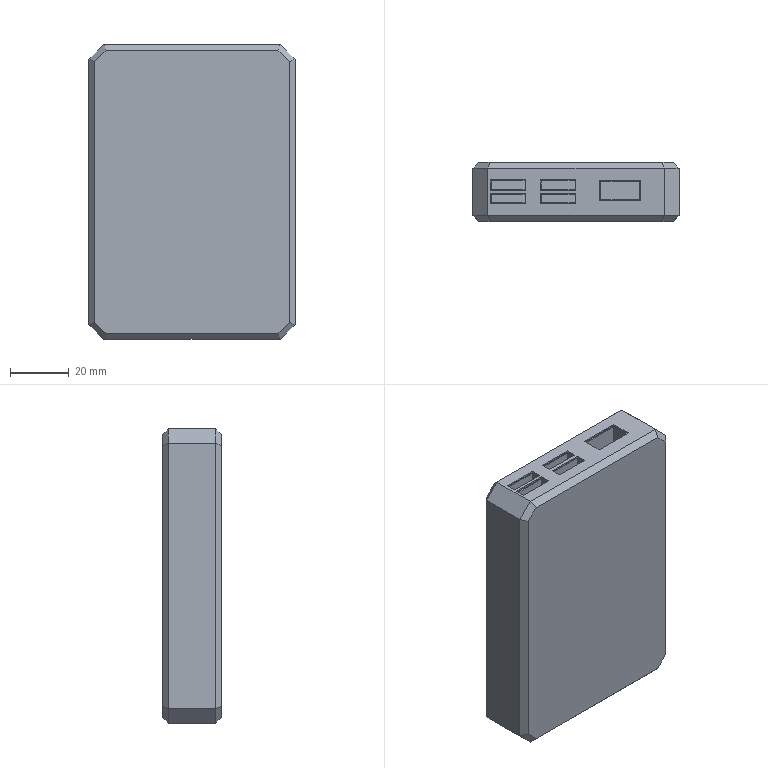Component | SolidWorks | WireBox-1 | 1 solid | 76 faces | box 70 x 20 x 100 mm | volume 135966 mm3 | plane 76
build123d program:
from build123d import *

# Parameters (mm, degrees)
BOSS_EXTRUDE1_DEPTH = 20
CHAMFER1_SIZE       = 2
SKETCH2_W           = 12
SKETCH2_H           = 3.5
SKETCH2_H_2         = 8
SKETCH2_W_2         = 14
SKETCH2_H_3         = 7
CUT_EXTRUDE1_DEPTH  = 8
SKETCH3_W           = 12
SKETCH3_H           = 1
BOSS_EXTRUDE2_DEPTH = 8
SKETCH4_W           = 14
SKETCH4_H           = 7
SKETCH4_W_2         = 13.2
SKETCH4_H_2         = 6.2
SKETCH4_W_3         = 12
SKETCH4_H_3         = 3.5
SKETCH4_W_4         = 11.4
SKETCH4_H_4         = 2.9
BOSS_EXTRUDE3_DEPTH = 7.5


with BuildPart() as part:
    # Sketch1 → Boss-Extrude1 (new body)
    with BuildSketch(Plane(origin=(0, 0, 0), x_dir=(1, 0, 0), z_dir=(0, 1, 0))):
        Polygon((-45, 35), (-50, 30), (-50, -30), (-45, -35), (45, -35), (50, -30), (50, 30), (45, 35), align=None)
    extrude(amount=BOSS_EXTRUDE1_DEPTH)

    # Chamfer1
    chamfer1_edges = [part.edges().sort_by_distance(p)[0] for p in [
        (47.5, 0, 32.5),
        (0, 0, 35),
        (-47.5, 0, 32.5),
        (-50, 0, 0),
        (0, 20, 35),
        (47.5, 20, 32.5),
        (50, 20, 0),
        (47.5, 20, -32.5),
        (0, 20, -35),
        (-47.5, 20, -32.5),
        (-50, 20, 0),
        (-47.5, 0, -32.5),
        (-47.5, 20, 32.5),
        (0, 0, -35),
        (47.5, 0, -32.5),
        (50, 0, 0),
    ]]
    chamfer(chamfer1_edges, length=CHAMFER1_SIZE)

    # Sketch2 → Cut-Extrude1 (cut)
    with BuildSketch(Plane(origin=(50, 0, 0), x_dir=(0, 0, -1), z_dir=(1, 0, 0))):
        with Locations((-23, 12.25)):
            Rectangle(SKETCH2_W, SKETCH2_H)
        with Locations((-23, 7.75)):
            Rectangle(SKETCH2_W, SKETCH2_H)
        with Locations((-6, 10)):
            Rectangle(SKETCH2_W, SKETCH2_H_2)
        with Locations((15, 10.427)):
            Rectangle(SKETCH2_W_2, SKETCH2_H_3)
    extrude(amount=-CUT_EXTRUDE1_DEPTH, mode=Mode.SUBTRACT)

    # Sketch3 → Boss-Extrude2 (add)
    with BuildSketch(Plane(origin=(42, 0, 0), x_dir=(0, 0, -1), z_dir=(1, 0, 0))):
        with Locations((-6, 10)):
            Rectangle(SKETCH3_W, SKETCH3_H)
    extrude(amount=BOSS_EXTRUDE2_DEPTH)

    # Sketch4 → Boss-Extrude3 (add)
    # profile 1 of 5: a face of its own
    with BuildSketch(Plane(origin=(42, 0, 0), x_dir=(0, 0, -1), z_dir=(1, 0, 0))):
        with Locations((15, 10.427)):
            Rectangle(SKETCH4_W, SKETCH4_H)
        with Locations((15, 10.427)):
            Rectangle(SKETCH4_W_2, SKETCH4_H_2, mode=Mode.SUBTRACT)
    # profile 2 of 5: a face of its own
    with BuildSketch(Plane(origin=(42, 0, 0), x_dir=(0, 0, -1), z_dir=(1, 0, 0))):
        with Locations((-6, 7.75)):
            Rectangle(SKETCH4_W_3, SKETCH4_H_3)
        with Locations((-6, 7.75)):
            Rectangle(SKETCH4_W_4, SKETCH4_H_4, mode=Mode.SUBTRACT)
    # profile 3 of 5: a face of its own
    with BuildSketch(Plane(origin=(42, 0, 0), x_dir=(0, 0, -1), z_dir=(1, 0, 0))):
        with Locations((-6, 12.25)):
            Rectangle(SKETCH4_W_3, SKETCH4_H_3)
        with Locations((-6, 12.25)):
            Rectangle(SKETCH4_W_4, SKETCH4_H_4, mode=Mode.SUBTRACT)
    # profile 4 of 5: a face of its own
    with BuildSketch(Plane(origin=(42, 0, 0), x_dir=(0, 0, -1), z_dir=(1, 0, 0))):
        with Locations((-23, 12.25)):
            Rectangle(SKETCH4_W_3, SKETCH4_H_3)
        with Locations((-23, 12.25)):
            Rectangle(SKETCH4_W_4, SKETCH4_H_4, mode=Mode.SUBTRACT)
    # profile 5 of 5: a face of its own
    with BuildSketch(Plane(origin=(42, 0, 0), x_dir=(0, 0, -1), z_dir=(1, 0, 0))):
        with Locations((-23, 7.75)):
            Rectangle(SKETCH4_W_3, SKETCH4_H_3)
        with Locations((-23, 7.75)):
            Rectangle(SKETCH4_W_4, SKETCH4_H_4, mode=Mode.SUBTRACT)
    extrude(amount=BOSS_EXTRUDE3_DEPTH)


solid = part.part

# Placed as in the assembly
solid = solid.moved(Location((-213.5, 598.5, 5), (0, -90, 0)))